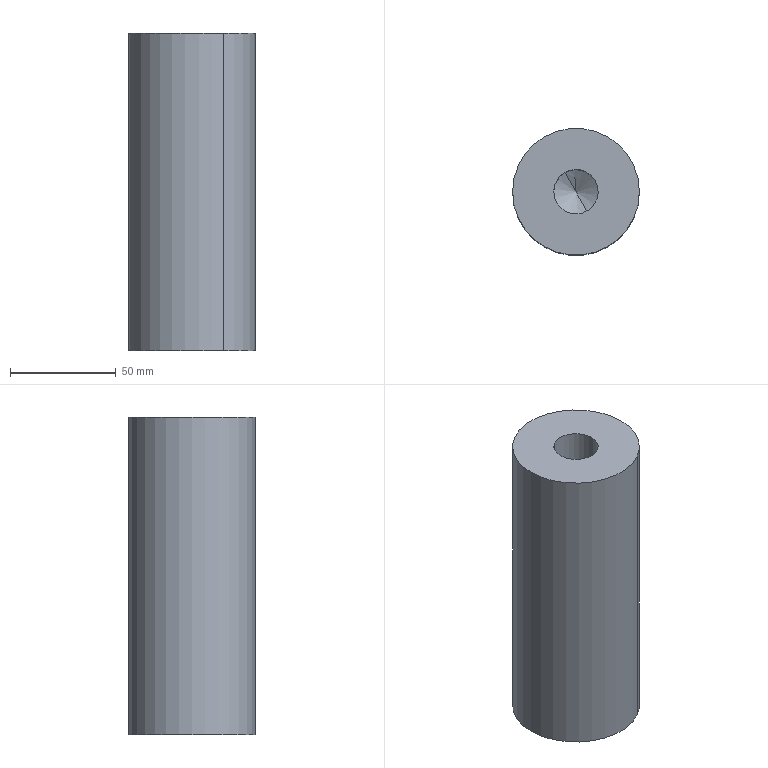Component | SolidWorks | KLHFH014_60HighGuideRod-4 | 1 solid | 12 faces | box 60 x 60 x 150 mm | volume 379017 mm3 | cylinder 6 | cone 4 | plane 2 | commonest cylinder face diameters 21 x4 60 x2 | material Plain Carbon Steel
build123d program:
from build123d import *

# Parameters (mm, degrees)
SKETCH1_R              = 30
BOSS_EXTRUDE1_DEPTH    = 75
M24_TAPPED_HOLE1_D     = 21
M24_TAPPED_HOLE1_DEPTH = 63
M24_TAPPED_HOLE1_TIP   = 6.309
M24_TAPPED_HOLE2_D     = 21
M24_TAPPED_HOLE2_DEPTH = 63
M24_TAPPED_HOLE2_TIP   = 6.309


with BuildPart() as part:
    # Sketch1 → Boss-Extrude1 (new, symmetric)
    with BuildSketch(Plane.XY):
        Circle(SKETCH1_R)
    extrude(amount=BOSS_EXTRUDE1_DEPTH, both=True)

    # M24 Tapped Hole1
    with Locations(Plane.XY.offset(75)):
        with Locations((0, 0)):
            Hole(M24_TAPPED_HOLE1_D / 2, depth=M24_TAPPED_HOLE1_DEPTH)
            with Locations((0, 0, -(M24_TAPPED_HOLE1_DEPTH + M24_TAPPED_HOLE1_TIP / 2))):  # 118° drill point
                Cone(0, M24_TAPPED_HOLE1_D / 2, M24_TAPPED_HOLE1_TIP, mode=Mode.SUBTRACT)

    # M24 Tapped Hole2
    with Locations(Plane(origin=(0, 0, -75), x_dir=(-1, 0, 0), z_dir=(0, 0, -1))):
        with Locations((0, 0)):
            Hole(M24_TAPPED_HOLE2_D / 2, depth=M24_TAPPED_HOLE2_DEPTH)
            with Locations((0, 0, -(M24_TAPPED_HOLE2_DEPTH + M24_TAPPED_HOLE2_TIP / 2))):  # 118° drill point
                Cone(0, M24_TAPPED_HOLE2_D / 2, M24_TAPPED_HOLE2_TIP, mode=Mode.SUBTRACT)


solid = part.part

# Placed as in the assembly
solid = solid.moved(Location((-110, 190.526, -82.5), (0, 0, 0)))
STEP:
#1=CARTESIAN_POINT('',(-4.537,7.859,-3.72));
#2=VERTEX_POINT('',#1);
#3=CARTESIAN_POINT('',(-4.124,7.143,-3.72));
#4=VERTEX_POINT('',#3);
#5=CARTESIAN_POINT('',(-4.331,7.501,-3.72));
#6=DIRECTION('',(0.,0.,-1.));
#7=DIRECTION('',(0.5,-0.866,0.));
#8=AXIS2_PLACEMENT_3D('',#5,#6,#7);
#9=CIRCLE('',#8,0.4134);
#10=EDGE_CURVE('',#2,#4,#9,.T.);
#11=ORIENTED_EDGE('',*,*,#10,.F.);
#12=CARTESIAN_POINT('',(-4.537,7.859,-6.201));
#13=VERTEX_POINT('',#12);
#14=CARTESIAN_POINT('',(-4.537,7.859,-6.201));
#15=DIRECTION('',(0.,0.,-1.));
#16=VECTOR('',#15,39.37);
#17=LINE('',#14,#16);
#18=EDGE_CURVE('',#2,#13,#17,.T.);
#19=ORIENTED_EDGE('',*,*,#18,.T.);
#20=CARTESIAN_POINT('',(-4.124,7.143,-6.201));
#21=VERTEX_POINT('',#20);
#22=CARTESIAN_POINT('',(-4.331,7.501,-6.201));
#23=DIRECTION('',(0.,0.,-1.));
#24=DIRECTION('',(0.5,-0.866,0.));
#25=AXIS2_PLACEMENT_3D('',#22,#23,#24);
#26=CIRCLE('',#25,0.4134);
#27=EDGE_CURVE('',#13,#21,#26,.T.);
#28=ORIENTED_EDGE('',*,*,#27,.T.);
#29=CARTESIAN_POINT('',(-4.124,7.143,-6.201));
#30=DIRECTION('',(0.,0.,-1.));
#31=VECTOR('',#30,39.37);
#32=LINE('',#29,#31);
#33=EDGE_CURVE('',#4,#21,#32,.T.);
#34=ORIENTED_EDGE('',*,*,#33,.F.);
#35=EDGE_LOOP('',(#11,#19,#28,#34));
#36=FACE_OUTER_BOUND('',#35,.T.);
#37=CARTESIAN_POINT('',(-4.331,7.501,-6.201));
#38=DIRECTION('',(0.,0.,-1.));
#39=DIRECTION('',(0.5,-0.866,0.));
#40=AXIS2_PLACEMENT_3D('',#37,#38,#39);
#41=CYLINDRICAL_SURFACE('',#40,0.4134);
#42=ADVANCED_FACE('',(#36),#41,.F.);
#43=CARTESIAN_POINT('',(-4.331,7.501,-3.472));
#44=VERTEX_POINT('',#43);
#45=CARTESIAN_POINT('',(-4.124,7.143,-3.72));
#46=DIRECTION('',(0.4286,-0.7423,-0.515));
#47=VECTOR('',#46,39.37);
#48=LINE('',#45,#47);
#49=EDGE_CURVE('',#44,#4,#48,.T.);
#50=ORIENTED_EDGE('',*,*,#49,.F.);
#51=CARTESIAN_POINT('',(-4.537,7.859,-3.72));
#52=DIRECTION('',(-0.4286,0.7423,-0.515));
#53=VECTOR('',#52,39.37);
#54=LINE('',#51,#53);
#55=EDGE_CURVE('',#44,#2,#54,.T.);
#56=ORIENTED_EDGE('',*,*,#55,.T.);
#57=ORIENTED_EDGE('',*,*,#10,.T.);
#58=EDGE_LOOP('',(#50,#56,#57));
#59=FACE_OUTER_BOUND('',#58,.T.);
#60=CARTESIAN_POINT('',(-4.331,7.501,-3.72));
#61=DIRECTION('',(0.,0.,-1.));
#62=DIRECTION('',(0.5,-0.866,0.));
#63=AXIS2_PLACEMENT_3D('',#60,#61,#62);
#64=CONICAL_SURFACE('',#63,0.4134,1.03);
#65=ADVANCED_FACE('',(#59),#64,.F.);
#66=CARTESIAN_POINT('',(-4.124,7.143,-2.776));
#67=VERTEX_POINT('',#66);
#68=CARTESIAN_POINT('',(-4.537,7.859,-2.776));
#69=VERTEX_POINT('',#68);
#70=CARTESIAN_POINT('',(-4.331,7.501,-2.776));
#71=DIRECTION('',(0.,0.,1.));
#72=DIRECTION('',(-0.5,0.866,0.));
#73=AXIS2_PLACEMENT_3D('',#70,#71,#72);
#74=CIRCLE('',#73,0.4134);
#75=EDGE_CURVE('',#67,#69,#74,.T.);
#76=ORIENTED_EDGE('',*,*,#75,.F.);
#77=CARTESIAN_POINT('',(-4.124,7.143,-0.2953));
#78=VERTEX_POINT('',#77);
#79=CARTESIAN_POINT('',(-4.124,7.143,-0.2953));
#80=DIRECTION('',(0.,0.,1.));
#81=VECTOR('',#80,39.37);
#82=LINE('',#79,#81);
#83=EDGE_CURVE('',#67,#78,#82,.T.);
#84=ORIENTED_EDGE('',*,*,#83,.T.);
#85=CARTESIAN_POINT('',(-4.537,7.859,-0.2953));
#86=VERTEX_POINT('',#85);
#87=CARTESIAN_POINT('',(-4.331,7.501,-0.2953));
#88=DIRECTION('',(0.,0.,1.));
#89=DIRECTION('',(-0.5,0.866,0.));
#90=AXIS2_PLACEMENT_3D('',#87,#88,#89);
#91=CIRCLE('',#90,0.4134);
#92=EDGE_CURVE('',#78,#86,#91,.T.);
#93=ORIENTED_EDGE('',*,*,#92,.T.);
#94=CARTESIAN_POINT('',(-4.537,7.859,-0.2953));
#95=DIRECTION('',(0.,0.,1.));
#96=VECTOR('',#95,39.37);
#97=LINE('',#94,#96);
#98=EDGE_CURVE('',#69,#86,#97,.T.);
#99=ORIENTED_EDGE('',*,*,#98,.F.);
#100=EDGE_LOOP('',(#76,#84,#93,#99));
#101=FACE_OUTER_BOUND('',#100,.T.);
#102=CARTESIAN_POINT('',(-4.331,7.501,-0.2953));
#103=DIRECTION('',(0.,0.,1.));
#104=DIRECTION('',(-0.5,0.866,0.));
#105=AXIS2_PLACEMENT_3D('',#102,#103,#104);
#106=CYLINDRICAL_SURFACE('',#105,0.4134);
#107=ADVANCED_FACE('',(#101),#106,.F.);
#108=CARTESIAN_POINT('',(-4.331,7.501,-3.024));
#109=VERTEX_POINT('',#108);
#110=CARTESIAN_POINT('',(-4.537,7.859,-2.776));
#111=DIRECTION('',(-0.4286,0.7423,0.515));
#112=VECTOR('',#111,39.37);
#113=LINE('',#110,#112);
#114=EDGE_CURVE('',#109,#69,#113,.T.);
#115=ORIENTED_EDGE('',*,*,#114,.F.);
#116=CARTESIAN_POINT('',(-4.124,7.143,-2.776));
#117=DIRECTION('',(0.4286,-0.7423,0.515));
#118=VECTOR('',#117,39.37);
#119=LINE('',#116,#118);
#120=EDGE_CURVE('',#109,#67,#119,.T.);
#121=ORIENTED_EDGE('',*,*,#120,.T.);
#122=ORIENTED_EDGE('',*,*,#75,.T.);
#123=EDGE_LOOP('',(#115,#121,#122));
#124=FACE_OUTER_BOUND('',#123,.T.);
#125=CARTESIAN_POINT('',(-4.331,7.501,-2.776));
#126=DIRECTION('',(0.,0.,1.));
#127=DIRECTION('',(-0.5,0.866,0.));
#128=AXIS2_PLACEMENT_3D('',#125,#126,#127);
#129=CONICAL_SURFACE('',#128,0.4134,1.03);
#130=ADVANCED_FACE('',(#124),#129,.F.);
#131=CARTESIAN_POINT('',(-4.921,8.524,-0.2953));
#132=VERTEX_POINT('',#131);
#133=CARTESIAN_POINT('',(-3.74,6.478,-0.2953));
#134=VERTEX_POINT('',#133);
#135=CARTESIAN_POINT('',(-4.331,7.501,-0.2953));
#136=DIRECTION('',(0.,0.,1.));
#137=DIRECTION('',(-0.5,0.866,0.));
#138=AXIS2_PLACEMENT_3D('',#135,#136,#137);
#139=CIRCLE('',#138,1.181);
#140=EDGE_CURVE('',#132,#134,#139,.T.);
#141=ORIENTED_EDGE('',*,*,#140,.F.);
#142=CARTESIAN_POINT('',(-4.921,8.524,-6.201));
#143=VERTEX_POINT('',#142);
#144=CARTESIAN_POINT('',(-4.921,8.524,-0.2953));
#145=DIRECTION('',(0.,0.,-1.));
#146=VECTOR('',#145,39.37);
#147=LINE('',#144,#146);
#148=EDGE_CURVE('',#132,#143,#147,.T.);
#149=ORIENTED_EDGE('',*,*,#148,.T.);
#150=CARTESIAN_POINT('',(-3.74,6.478,-6.201));
#151=VERTEX_POINT('',#150);
#152=CARTESIAN_POINT('',(-4.331,7.501,-6.201));
#153=DIRECTION('',(0.,0.,1.));
#154=DIRECTION('',(-0.5,0.866,0.));
#155=AXIS2_PLACEMENT_3D('',#152,#153,#154);
#156=CIRCLE('',#155,1.181);
#157=EDGE_CURVE('',#143,#151,#156,.T.);
#158=ORIENTED_EDGE('',*,*,#157,.T.);
#159=CARTESIAN_POINT('',(-3.74,6.478,-0.2953));
#160=DIRECTION('',(0.,0.,-1.));
#161=VECTOR('',#160,39.37);
#162=LINE('',#159,#161);
#163=EDGE_CURVE('',#134,#151,#162,.T.);
#164=ORIENTED_EDGE('',*,*,#163,.F.);
#165=EDGE_LOOP('',(#141,#149,#158,#164));
#166=FACE_OUTER_BOUND('',#165,.T.);
#167=CARTESIAN_POINT('',(-4.331,7.501,-0.2953));
#168=DIRECTION('',(0.,0.,-1.));
#169=DIRECTION('',(0.5,-0.866,0.));
#170=AXIS2_PLACEMENT_3D('',#167,#168,#169);
#171=CYLINDRICAL_SURFACE('',#170,1.181);
#172=ADVANCED_FACE('',(#166),#171,.T.);
#173=ORIENTED_EDGE('',*,*,#148,.F.);
#174=CARTESIAN_POINT('',(-4.331,7.501,-0.2953));
#175=DIRECTION('',(0.,0.,1.));
#176=DIRECTION('',(-0.5,0.866,0.));
#177=AXIS2_PLACEMENT_3D('',#174,#175,#176);
#178=CIRCLE('',#177,1.181);
#179=EDGE_CURVE('',#134,#132,#178,.T.);
#180=ORIENTED_EDGE('',*,*,#179,.F.);
#181=ORIENTED_EDGE('',*,*,#163,.T.);
#182=CARTESIAN_POINT('',(-4.331,7.501,-6.201));
#183=DIRECTION('',(0.,0.,1.));
#184=DIRECTION('',(-0.5,0.866,0.));
#185=AXIS2_PLACEMENT_3D('',#182,#183,#184);
#186=CIRCLE('',#185,1.181);
#187=EDGE_CURVE('',#151,#143,#186,.T.);
#188=ORIENTED_EDGE('',*,*,#187,.T.);
#189=EDGE_LOOP('',(#173,#180,#181,#188));
#190=FACE_OUTER_BOUND('',#189,.T.);
#191=CARTESIAN_POINT('',(-4.331,7.501,-0.2953));
#192=DIRECTION('',(0.,0.,-1.));
#193=DIRECTION('',(0.5,-0.866,0.));
#194=AXIS2_PLACEMENT_3D('',#191,#192,#193);
#195=CYLINDRICAL_SURFACE('',#194,1.181);
#196=ADVANCED_FACE('',(#190),#195,.T.);
#197=CARTESIAN_POINT('',(-4.331,7.501,-0.2953));
#198=DIRECTION('',(0.,0.,1.));
#199=DIRECTION('',(-0.5,0.866,0.));
#200=AXIS2_PLACEMENT_3D('',#197,#198,#199);
#201=CIRCLE('',#200,0.4134);
#202=EDGE_CURVE('',#86,#78,#201,.T.);
#203=ORIENTED_EDGE('',*,*,#202,.F.);
#204=ORIENTED_EDGE('',*,*,#92,.F.);
#205=EDGE_LOOP('',(#203,#204));
#206=FACE_BOUND('',#205,.T.);
#207=ORIENTED_EDGE('',*,*,#179,.T.);
#208=ORIENTED_EDGE('',*,*,#140,.T.);
#209=EDGE_LOOP('',(#207,#208));
#210=FACE_OUTER_BOUND('',#209,.T.);
#211=CARTESIAN_POINT('',(-4.331,7.501,-0.2953));
#212=DIRECTION('',(0.,0.,1.));
#213=DIRECTION('',(-0.5,0.866,0.));
#214=AXIS2_PLACEMENT_3D('',#211,#212,#213);
#215=PLANE('',#214);
#216=ADVANCED_FACE('',(#206,#210),#215,.T.);
#217=CARTESIAN_POINT('',(-4.331,7.501,-6.201));
#218=DIRECTION('',(0.,0.,-1.));
#219=DIRECTION('',(0.5,-0.866,0.));
#220=AXIS2_PLACEMENT_3D('',#217,#218,#219);
#221=CIRCLE('',#220,0.4134);
#222=EDGE_CURVE('',#21,#13,#221,.T.);
#223=ORIENTED_EDGE('',*,*,#222,.F.);
#224=ORIENTED_EDGE('',*,*,#27,.F.);
#225=EDGE_LOOP('',(#223,#224));
#226=FACE_BOUND('',#225,.T.);
#227=ORIENTED_EDGE('',*,*,#187,.F.);
#228=ORIENTED_EDGE('',*,*,#157,.F.);
#229=EDGE_LOOP('',(#227,#228));
#230=FACE_OUTER_BOUND('',#229,.T.);
#231=CARTESIAN_POINT('',(-4.331,7.501,-6.201));
#232=DIRECTION('',(0.,0.,1.));
#233=DIRECTION('',(-0.5,0.866,0.));
#234=AXIS2_PLACEMENT_3D('',#231,#232,#233);
#235=PLANE('',#234);
#236=ADVANCED_FACE('',(#226,#230),#235,.F.);
#237=ORIENTED_EDGE('',*,*,#120,.F.);
#238=ORIENTED_EDGE('',*,*,#114,.T.);
#239=CARTESIAN_POINT('',(-4.331,7.501,-2.776));
#240=DIRECTION('',(0.,0.,1.));
#241=DIRECTION('',(-0.5,0.866,0.));
#242=AXIS2_PLACEMENT_3D('',#239,#240,#241);
#243=CIRCLE('',#242,0.4134);
#244=EDGE_CURVE('',#69,#67,#243,.T.);
#245=ORIENTED_EDGE('',*,*,#244,.T.);
#246=EDGE_LOOP('',(#237,#238,#245));
#247=FACE_OUTER_BOUND('',#246,.T.);
#248=CARTESIAN_POINT('',(-4.331,7.501,-2.776));
#249=DIRECTION('',(0.,0.,1.));
#250=DIRECTION('',(-0.5,0.866,0.));
#251=AXIS2_PLACEMENT_3D('',#248,#249,#250);
#252=CONICAL_SURFACE('',#251,0.4134,1.03);
#253=ADVANCED_FACE('',(#247),#252,.F.);
#254=ORIENTED_EDGE('',*,*,#83,.F.);
#255=ORIENTED_EDGE('',*,*,#244,.F.);
#256=ORIENTED_EDGE('',*,*,#98,.T.);
#257=ORIENTED_EDGE('',*,*,#202,.T.);
#258=EDGE_LOOP('',(#254,#255,#256,#257));
#259=FACE_OUTER_BOUND('',#258,.T.);
#260=CARTESIAN_POINT('',(-4.331,7.501,-0.2953));
#261=DIRECTION('',(0.,0.,1.));
#262=DIRECTION('',(-0.5,0.866,0.));
#263=AXIS2_PLACEMENT_3D('',#260,#261,#262);
#264=CYLINDRICAL_SURFACE('',#263,0.4134);
#265=ADVANCED_FACE('',(#259),#264,.F.);
#266=ORIENTED_EDGE('',*,*,#55,.F.);
#267=ORIENTED_EDGE('',*,*,#49,.T.);
#268=CARTESIAN_POINT('',(-4.331,7.501,-3.72));
#269=DIRECTION('',(0.,0.,-1.));
#270=DIRECTION('',(0.5,-0.866,0.));
#271=AXIS2_PLACEMENT_3D('',#268,#269,#270);
#272=CIRCLE('',#271,0.4134);
#273=EDGE_CURVE('',#4,#2,#272,.T.);
#274=ORIENTED_EDGE('',*,*,#273,.T.);
#275=EDGE_LOOP('',(#266,#267,#274));
#276=FACE_OUTER_BOUND('',#275,.T.);
#277=CARTESIAN_POINT('',(-4.331,7.501,-3.72));
#278=DIRECTION('',(0.,0.,-1.));
#279=DIRECTION('',(0.5,-0.866,0.));
#280=AXIS2_PLACEMENT_3D('',#277,#278,#279);
#281=CONICAL_SURFACE('',#280,0.4134,1.03);
#282=ADVANCED_FACE('',(#276),#281,.F.);
#283=ORIENTED_EDGE('',*,*,#18,.F.);
#284=ORIENTED_EDGE('',*,*,#273,.F.);
#285=ORIENTED_EDGE('',*,*,#33,.T.);
#286=ORIENTED_EDGE('',*,*,#222,.T.);
#287=EDGE_LOOP('',(#283,#284,#285,#286));
#288=FACE_OUTER_BOUND('',#287,.T.);
#289=CARTESIAN_POINT('',(-4.331,7.501,-6.201));
#290=DIRECTION('',(0.,0.,-1.));
#291=DIRECTION('',(0.5,-0.866,0.));
#292=AXIS2_PLACEMENT_3D('',#289,#290,#291);
#293=CYLINDRICAL_SURFACE('',#292,0.4134);
#294=ADVANCED_FACE('',(#288),#293,.F.);
#295=CLOSED_SHELL('',(#42,#65,#107,#130,#172,#196,#216,#236,#253,#265,#282,#294));
#296=MANIFOLD_SOLID_BREP('',#295);
#297=CARTESIAN_POINT('',(0.,0.,0.));
#298=DIRECTION('',(0.,0.,1.));
#299=DIRECTION('',(1.,0.,0.));
#300=AXIS2_PLACEMENT_3D('',#297,#298,#299);
#301=(LENGTH_UNIT()NAMED_UNIT(*)SI_UNIT($,.METRE.));
#302=LENGTH_MEASURE_WITH_UNIT(LENGTH_MEASURE(0.0254),#301);
#303=DIMENSIONAL_EXPONENTS(1.,0.,0.,0.,0.,0.,0.);
#304=(CONVERSION_BASED_UNIT('',#302)LENGTH_UNIT()NAMED_UNIT(#303));
#305=UNCERTAINTY_MEASURE_WITH_UNIT(LENGTH_MEASURE(0.00001),#304,'','');
#306=(NAMED_UNIT(*)PLANE_ANGLE_UNIT()SI_UNIT($,.RADIAN.));
#307=(NAMED_UNIT(*)SI_UNIT($,.STERADIAN.)SOLID_ANGLE_UNIT());
#308=(GEOMETRIC_REPRESENTATION_CONTEXT(3)GLOBAL_UNCERTAINTY_ASSIGNED_CONTEXT((#305))GLOBAL_UNIT_ASSIGNED_CONTEXT((#304,#306,#307))REPRESENTATION_CONTEXT('',''));
#309=ADVANCED_BREP_SHAPE_REPRESENTATION('',(#296,#300),#308);
#310=COLOUR_RGB('',0.7922,0.8196,0.9333);
#311=FILL_AREA_STYLE_COLOUR('',#310);
#312=FILL_AREA_STYLE('',(#311));
#313=SURFACE_STYLE_FILL_AREA(#312);
#314=SURFACE_SIDE_STYLE('',(#313));
#315=SURFACE_STYLE_USAGE(.BOTH.,#314);
#316=PRESENTATION_STYLE_ASSIGNMENT((#315));
#317=STYLED_ITEM('',(#316),#296);
#318=PRESENTATION_LAYER_ASSIGNMENT('','',(#317));
#319=(LENGTH_UNIT()NAMED_UNIT(*)SI_UNIT($,.METRE.));
#320=LENGTH_MEASURE_WITH_UNIT(LENGTH_MEASURE(0.0254),#319);
#321=DIMENSIONAL_EXPONENTS(1.,0.,0.,0.,0.,0.,0.);
#322=(CONVERSION_BASED_UNIT('',#320)LENGTH_UNIT()NAMED_UNIT(#321));
#323=UNCERTAINTY_MEASURE_WITH_UNIT(LENGTH_MEASURE(0.00001),#322,'','');
#324=(NAMED_UNIT(*)PLANE_ANGLE_UNIT()SI_UNIT($,.RADIAN.));
#325=(NAMED_UNIT(*)SI_UNIT($,.STERADIAN.)SOLID_ANGLE_UNIT());
#326=(GEOMETRIC_REPRESENTATION_CONTEXT(3)GLOBAL_UNCERTAINTY_ASSIGNED_CONTEXT((#323))GLOBAL_UNIT_ASSIGNED_CONTEXT((#322,#324,#325))REPRESENTATION_CONTEXT('',''));
#327=MECHANICAL_DESIGN_GEOMETRIC_PRESENTATION_REPRESENTATION('',(#317),#326);